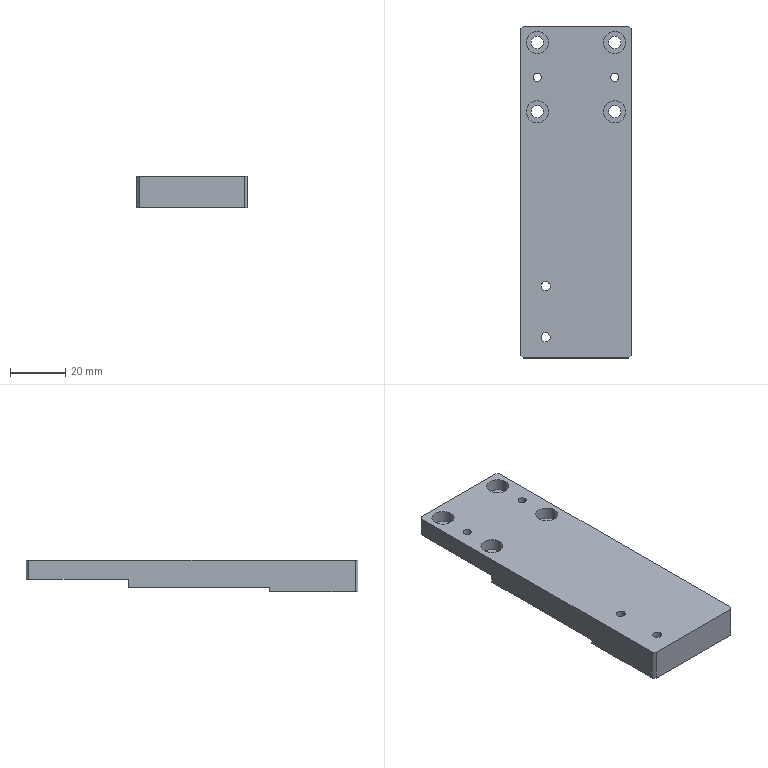Component | SolidWorks | 002MaterialPickingModuleA-1_004SidePlugModule-1_J-016-2 | 1 solid | 42 faces | box 40 x 120 x 11.5 mm | volume 44116 mm3 | cylinder 24 | plane 18 | commonest cylinder face diameters 8 x8 4.5 x8 3.3 x4 3 x4 | material 45
build123d program:
from build123d import *

# Parameters (mm, degrees)
SKETCH2_W                                       = 40
SKETCH2_H                                       = 120
BOSS_EXTRUDE1_DEPTH                             = 10
SKETCH3_W                                       = 40
SKETCH3_H                                       = 37
CUT_EXTRUDE1_DEPTH                              = 3
M4_HEX_SOCKET_HEAD_CAP_SCREW_CBORE1_D           = 4.5
M4_HEX_SOCKET_HEAD_CAP_SCREW_CBORE1_CBORE_D     = 8
M4_HEX_SOCKET_HEAD_CAP_SCREW_CBORE1_CBORE_DEPTH = 4.4
SIZE_MM_DOWEL_PIN_HOLE1_D                       = 3
SKETCH8_W                                       = 40
SKETCH8_H                                       = 32
BOSS_EXTRUDE2_DEPTH                             = 1.5
M4_TAPPED_HOLE1_D                               = 3.3
CHAMFER1_SIZE                                   = 1


with BuildPart() as part:
    # Sketch2 → Boss-Extrude1 (new body)
    with BuildSketch(Plane.XY):
        Rectangle(SKETCH2_W, SKETCH2_H)
    extrude(amount=BOSS_EXTRUDE1_DEPTH)

    # Sketch3 → Cut-Extrude1 (cut)
    with BuildSketch(Plane(origin=(0, 0, 0), x_dir=(-1, 0, 0), z_dir=(0, 0, -1))):
        with Locations((0, 41.5)):
            Rectangle(SKETCH3_W, SKETCH3_H)
    extrude(amount=-CUT_EXTRUDE1_DEPTH, mode=Mode.SUBTRACT)

    # M4 Hex Socket Head Cap Screw CBORE1 (through all)
    with Locations(Plane.XY.offset(10)):
        with Locations((-14, 54), (-14, 29), (14, 54), (14, 29)):
            CounterBoreHole(M4_HEX_SOCKET_HEAD_CAP_SCREW_CBORE1_D / 2, M4_HEX_SOCKET_HEAD_CAP_SCREW_CBORE1_CBORE_D / 2, M4_HEX_SOCKET_HEAD_CAP_SCREW_CBORE1_CBORE_DEPTH)

    # Size mm Dowel Pin Hole1 (through all)
    with Locations(Plane.XY.offset(10)):
        with Locations((-14, 41.5), (14, 41.5)):
            Hole(SIZE_MM_DOWEL_PIN_HOLE1_D / 2)

    # Sketch8 → Boss-Extrude2 (add)
    with BuildSketch(Plane(origin=(0, 0, 0), x_dir=(-1, 0, 0), z_dir=(0, 0, -1))):
        with Locations((0, -44)):
            Rectangle(SKETCH8_W, SKETCH8_H)
    extrude(amount=BOSS_EXTRUDE2_DEPTH)

    # M4 Tapped Hole1 (through all)
    with Locations(Plane(origin=(0, 0, -1.5), x_dir=(-1, 0, 0), z_dir=(0, 0, -1))):
        with Locations((11, -34), (11, -52.5)):
            Hole(M4_TAPPED_HOLE1_D / 2)

    # Chamfer1
    chamfer1_edges = [part.edges().sort_by_distance(p)[0] for p in [
        (-20, 60, 6.5),
        (20, 60, 6.5),
        (20, -60, 4.25),
        (-20, -60, 4.25),
    ]]
    chamfer(chamfer1_edges, length=CHAMFER1_SIZE)


solid = part.part

# Placed as in the assembly
solid = solid.moved(Location((220.325, 268.019, 477.731), (0, 0, 0)))